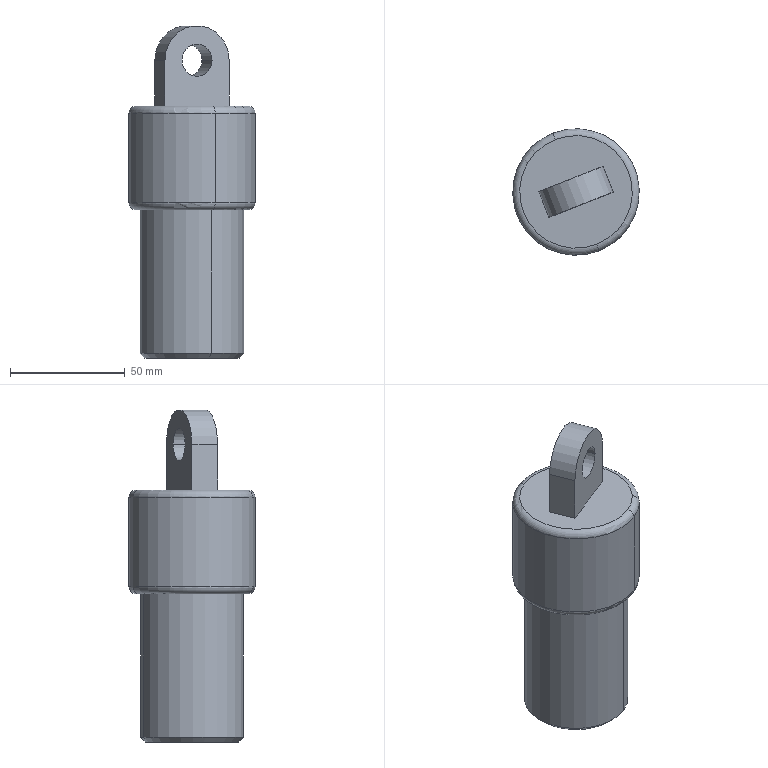Component | SolidWorks | KLHFH006_18LocatingPinFixingSeat-1 | 1 solid | 43 faces | box 55 x 55 x 144.5 mm | volume 215151 mm3 | cylinder 19 | cone 12 | plane 8 | torus 4 | commonest cylinder face diameters 3.3 x8 5 x2 12 x2 14 x2 55 x2 45 x2 30 x1 | material Plain Carbon Steel
build123d program:
from build123d import *

# Parameters (mm, degrees)
SKETCH2_R             = 22.5
BOSS_EXTRUDE1_DEPTH   = 64.5
SKETCH3_R             = 27.5
BOSS_EXTRUDE2_DEPTH   = 45
SKETCH5_W             = 12
SKETCH5_H             = 30
BOSS_EXTRUDE3_DEPTH   = 35
CUT_EXTRUDE1_DEPTH    = 151.86
SKETCH7_R             = 7
CUT_EXTRUDE2_DEPTH    = 151.86
SKETCH8_R             = 6
CUT_EXTRUDE3_DEPTH    = 15
M6_TAPPED_HOLE1_D     = 5
M6_TAPPED_HOLE1_DEPTH = 25
M6_TAPPED_HOLE1_TIP   = 1.502
FILLET1_R             = 3
CHAMFER1_SIZE         = 2
CIRPATTERN1_COUNT     = 4


with BuildPart() as part:
    # Sketch2 → Boss-Extrude1 (new body)
    with BuildSketch(Plane.XY):
        Circle(SKETCH2_R)
    extrude(amount=BOSS_EXTRUDE1_DEPTH)

    # Sketch3 → Boss-Extrude2 (add)
    with BuildSketch(Plane.XY.offset(64.5)):
        with Locations(Location((0, 0, 0), (0, 0, 180))):
            Circle(SKETCH3_R)
    extrude(amount=BOSS_EXTRUDE2_DEPTH)

    # Sketch5 → Boss-Extrude3 (add)
    with BuildSketch(Plane.XY.offset(109.5)):
        Rectangle(SKETCH5_W, SKETCH5_H)
    extrude(amount=BOSS_EXTRUDE3_DEPTH)

    # Sketch6 → Cut-Extrude1 (cut, through all)
    with BuildSketch(Plane(origin=(6, 0, 0), x_dir=(0, 0, -1), z_dir=(1, 0, 0))):
        with BuildLine():
            Line((-129.5, 15), (-227.389, 15))
            Line((-227.389, 15), (-227.389, -15))
            Line((-227.389, -15), (-129.5, -15))
            ThreePointArc((-129.5, -15), (-144.5, 0), (-129.5, 15))
        make_face()
    extrude(amount=-CUT_EXTRUDE1_DEPTH, mode=Mode.SUBTRACT)

    # Sketch7 → Cut-Extrude2 (cut, through all)
    with BuildSketch(Plane(origin=(6, 0, 0), x_dir=(0, 0, -1), z_dir=(1, 0, 0))):
        with Locations(Location((-129.5, 0, 0), (0, 0, 90))):
            Circle(SKETCH7_R)
    extrude(amount=-CUT_EXTRUDE2_DEPTH, mode=Mode.SUBTRACT)

    # Sketch8 → Cut-Extrude3 (cut)
    with BuildSketch(Plane(origin=(0, 0, 0), x_dir=(-1, 0, 0), z_dir=(0, 0, -1))):
        Circle(SKETCH8_R)
    extrude(amount=-CUT_EXTRUDE3_DEPTH, mode=Mode.SUBTRACT)

    # M6 Tapped Hole1
    with Locations(Plane(origin=(0, 0, 15), x_dir=(-1, 0, 0), z_dir=(0, 0, -1))):
        with Locations((0, 0)):
            Hole(M6_TAPPED_HOLE1_D / 2, depth=M6_TAPPED_HOLE1_DEPTH)
            with Locations((0, 0, -(M6_TAPPED_HOLE1_DEPTH + M6_TAPPED_HOLE1_TIP / 2))):  # 118° drill point
                Cone(0, M6_TAPPED_HOLE1_D / 2, M6_TAPPED_HOLE1_TIP, mode=Mode.SUBTRACT)

    # Fillet1
    fillet1_edges = [part.edges().sort_by_distance(p)[0] for p in [
        (27.5, 0, 64.5),
        (27.5, 0, 109.5),
    ]]
    fillet(fillet1_edges, radius=FILLET1_R)

    # Chamfer1
    chamfer1_edges = [part.edges().sort_by_distance(p)[0] for p in [
        (-22.5, 0, 0),
    ]]
    chamfer(chamfer1_edges, length=CHAMFER1_SIZE)

    # Sketch14 → M4 Tapped Hole1 (revolve, cut)
    with BuildSketch(Plane(origin=(0, 14, 0), x_dir=(0, 1, 0), z_dir=(1, 0, 0))):
        Polygon((0, 0), (0, 24.491), (1.65, 23.5), (1.65, 0), align=None)
    m4_tapped_hole1 = revolve(axis=Axis((0, 14, -6.35), (0, 0, 1)), mode=Mode.SUBTRACT)

    # CirPattern1: M4 Tapped Hole1 ×4 about axis
    cirpattern1_axis = Axis((0, 0, 0), (0, 0, 1))
    for i in range(1, CIRPATTERN1_COUNT):
        add(m4_tapped_hole1.rotate(cirpattern1_axis, i * 360 / CIRPATTERN1_COUNT), mode=Mode.SUBTRACT)


solid = part.part

# Placed as in the assembly
solid = solid.moved(Location((91, 157.617, -335.5), (0, 0, 111.556)))